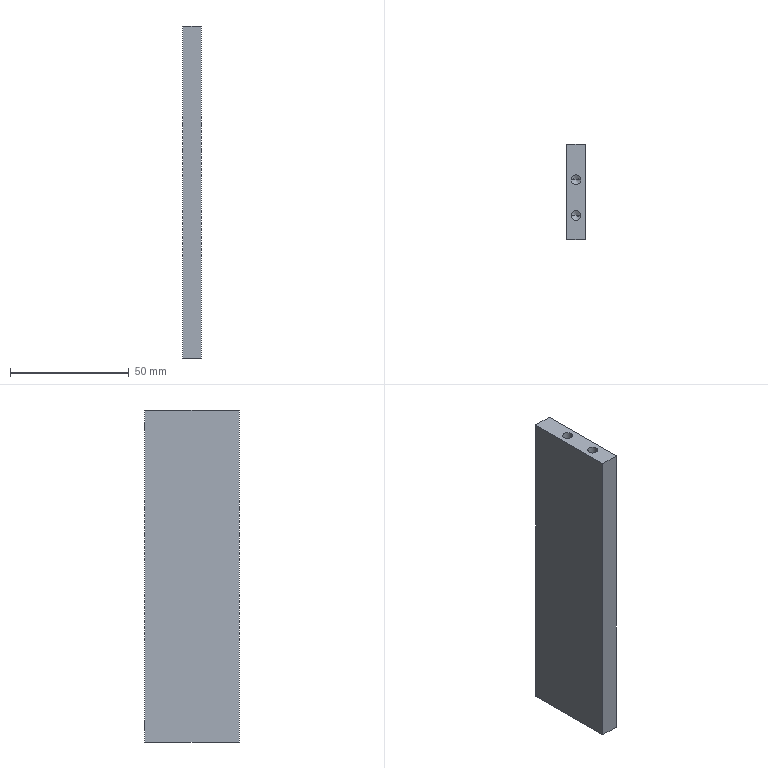Component | SolidWorks | FrameFrontMatchingPlate.1-1 | 1 solid | 30 faces | box 8 x 40 x 140 mm | volume 43911 mm3 | cylinder 12 | cone 12 | plane 6 | commonest cylinder face diameters 4.2 x8 3.3 x4
build123d program:
from build123d import *

# Parameters (mm, degrees)
SKETCH1_W             = 140
SKETCH1_H             = 40
BOSS_EXTRUDE1_DEPTH   = 8
M5_TAPPED_HOLE1_D     = 4.2
M5_TAPPED_HOLE1_DEPTH = 12.4
M5_TAPPED_HOLE1_TIP   = 1.262
M5_TAPPED_HOLE2_D     = 4.2
M5_TAPPED_HOLE2_DEPTH = 12.4
M5_TAPPED_HOLE2_TIP   = 1.262
M4_TAPPED_HOLE1_D     = 3.3
M4_TAPPED_HOLE1_DEPTH = 10.1
M4_TAPPED_HOLE1_TIP   = 0.9914


with BuildPart() as part:
    # Sketch1 → Boss-Extrude1 (new body)
    with BuildSketch(Plane.XY):
        Rectangle(SKETCH1_W, SKETCH1_H)
    extrude(amount=BOSS_EXTRUDE1_DEPTH)

    # M5 Tapped Hole1
    with Locations(Plane(origin=(70, 0, 0), x_dir=(0, 0, -1), z_dir=(1, 0, 0))):
        with Locations((-4, 5), (-4, -10)):
            Hole(M5_TAPPED_HOLE1_D / 2, depth=M5_TAPPED_HOLE1_DEPTH)
            with Locations((0, 0, -(M5_TAPPED_HOLE1_DEPTH + M5_TAPPED_HOLE1_TIP / 2))):  # 118° drill point
                Cone(0, M5_TAPPED_HOLE1_D / 2, M5_TAPPED_HOLE1_TIP, mode=Mode.SUBTRACT)

    # M5 Tapped Hole2
    with Locations(Plane.ZY.offset(70)):
        with Locations((4, 5), (4, -10)):
            Hole(M5_TAPPED_HOLE2_D / 2, depth=M5_TAPPED_HOLE2_DEPTH)
            with Locations((0, 0, -(M5_TAPPED_HOLE2_DEPTH + M5_TAPPED_HOLE2_TIP / 2))):  # 118° drill point
                Cone(0, M5_TAPPED_HOLE2_D / 2, M5_TAPPED_HOLE2_TIP, mode=Mode.SUBTRACT)

    # M4 Tapped Hole1
    with Locations(Plane(origin=(0, 20, 0), x_dir=(-1, 0, 0), z_dir=(0, 1, 0))):
        with Locations((63, 4), (-63, 4)):
            Hole(M4_TAPPED_HOLE1_D / 2, depth=M4_TAPPED_HOLE1_DEPTH)
            with Locations((0, 0, -(M4_TAPPED_HOLE1_DEPTH + M4_TAPPED_HOLE1_TIP / 2))):  # 118° drill point
                Cone(0, M4_TAPPED_HOLE1_D / 2, M4_TAPPED_HOLE1_TIP, mode=Mode.SUBTRACT)


solid = part.part

# Placed as in the assembly
solid = solid.moved(Location((13, 126.5, 0), (0, 90, 0)))
STEP:
#1=COLOUR_RGB('',0.7922,0.8196,0.9333);
#2=FILL_AREA_STYLE_COLOUR('',#1);
#3=FILL_AREA_STYLE('',(#2));
#4=SURFACE_STYLE_FILL_AREA(#3);
#5=SURFACE_SIDE_STYLE('',(#4));
#6=SURFACE_STYLE_USAGE(.BOTH.,#5);
#7=PRESENTATION_STYLE_ASSIGNMENT((#6));
#8=CARTESIAN_POINT('',(0.6043,5.37,2.48));
#9=VERTEX_POINT('',#8);
#10=CARTESIAN_POINT('',(0.7343,5.37,2.48));
#11=VERTEX_POINT('',#10);
#12=CARTESIAN_POINT('',(0.6693,5.37,2.48));
#13=DIRECTION('',(0.,1.,0.));
#14=DIRECTION('',(1.,0.,0.));
#15=AXIS2_PLACEMENT_3D('',#12,#13,#14);
#16=CIRCLE('',#15,0.06496);
#17=EDGE_CURVE('',#9,#11,#16,.T.);
#18=ORIENTED_EDGE('',*,*,#17,.F.);
#19=CARTESIAN_POINT('',(0.6043,5.768,2.48));
#20=VERTEX_POINT('',#19);
#21=CARTESIAN_POINT('',(0.6043,5.768,2.48));
#22=DIRECTION('',(0.,1.,0.));
#23=VECTOR('',#22,39.37);
#24=LINE('',#21,#23);
#25=EDGE_CURVE('',#9,#20,#24,.T.);
#26=ORIENTED_EDGE('',*,*,#25,.T.);
#27=CARTESIAN_POINT('',(0.7343,5.768,2.48));
#28=VERTEX_POINT('',#27);
#29=CARTESIAN_POINT('',(0.6693,5.768,2.48));
#30=DIRECTION('',(0.,1.,0.));
#31=DIRECTION('',(1.,0.,0.));
#32=AXIS2_PLACEMENT_3D('',#29,#30,#31);
#33=CIRCLE('',#32,0.06496);
#34=EDGE_CURVE('',#20,#28,#33,.T.);
#35=ORIENTED_EDGE('',*,*,#34,.T.);
#36=CARTESIAN_POINT('',(0.7343,5.768,2.48));
#37=DIRECTION('',(0.,1.,0.));
#38=VECTOR('',#37,39.37);
#39=LINE('',#36,#38);
#40=EDGE_CURVE('',#11,#28,#39,.T.);
#41=ORIENTED_EDGE('',*,*,#40,.F.);
#42=EDGE_LOOP('',(#18,#26,#35,#41));
#43=FACE_OUTER_BOUND('',#42,.T.);
#44=CARTESIAN_POINT('',(0.6693,5.768,2.48));
#45=DIRECTION('',(0.,1.,0.));
#46=DIRECTION('',(1.,0.,0.));
#47=AXIS2_PLACEMENT_3D('',#44,#45,#46);
#48=CYLINDRICAL_SURFACE('',#47,0.06496);
#49=ADVANCED_FACE('',(#43),#48,.F.);
#50=CARTESIAN_POINT('',(0.6693,5.331,2.48));
#51=VERTEX_POINT('',#50);
#52=CARTESIAN_POINT('',(0.7343,5.37,2.48));
#53=DIRECTION('',(0.8572,0.515,0.));
#54=VECTOR('',#53,39.37);
#55=LINE('',#52,#54);
#56=EDGE_CURVE('',#51,#11,#55,.T.);
#57=ORIENTED_EDGE('',*,*,#56,.F.);
#58=CARTESIAN_POINT('',(0.6043,5.37,2.48));
#59=DIRECTION('',(-0.8572,0.515,-0.));
#60=VECTOR('',#59,39.37);
#61=LINE('',#58,#60);
#62=EDGE_CURVE('',#51,#9,#61,.T.);
#63=ORIENTED_EDGE('',*,*,#62,.T.);
#64=ORIENTED_EDGE('',*,*,#17,.T.);
#65=EDGE_LOOP('',(#57,#63,#64));
#66=FACE_OUTER_BOUND('',#65,.T.);
#67=CARTESIAN_POINT('',(0.6693,5.37,2.48));
#68=DIRECTION('',(0.,1.,0.));
#69=DIRECTION('',(1.,0.,0.));
#70=AXIS2_PLACEMENT_3D('',#67,#68,#69);
#71=CONICAL_SURFACE('',#70,0.06496,1.03);
#72=ADVANCED_FACE('',(#66),#71,.F.);
#73=CARTESIAN_POINT('',(0.6043,5.37,-2.48));
#74=VERTEX_POINT('',#73);
#75=CARTESIAN_POINT('',(0.7343,5.37,-2.48));
#76=VERTEX_POINT('',#75);
#77=CARTESIAN_POINT('',(0.6693,5.37,-2.48));
#78=DIRECTION('',(0.,1.,0.));
#79=DIRECTION('',(1.,0.,0.));
#80=AXIS2_PLACEMENT_3D('',#77,#78,#79);
#81=CIRCLE('',#80,0.06496);
#82=EDGE_CURVE('',#74,#76,#81,.T.);
#83=ORIENTED_EDGE('',*,*,#82,.F.);
#84=CARTESIAN_POINT('',(0.6043,5.768,-2.48));
#85=VERTEX_POINT('',#84);
#86=CARTESIAN_POINT('',(0.6043,5.768,-2.48));
#87=DIRECTION('',(0.,1.,0.));
#88=VECTOR('',#87,39.37);
#89=LINE('',#86,#88);
#90=EDGE_CURVE('',#74,#85,#89,.T.);
#91=ORIENTED_EDGE('',*,*,#90,.T.);
#92=CARTESIAN_POINT('',(0.7343,5.768,-2.48));
#93=VERTEX_POINT('',#92);
#94=CARTESIAN_POINT('',(0.6693,5.768,-2.48));
#95=DIRECTION('',(0.,1.,0.));
#96=DIRECTION('',(1.,0.,0.));
#97=AXIS2_PLACEMENT_3D('',#94,#95,#96);
#98=CIRCLE('',#97,0.06496);
#99=EDGE_CURVE('',#85,#93,#98,.T.);
#100=ORIENTED_EDGE('',*,*,#99,.T.);
#101=CARTESIAN_POINT('',(0.7343,5.768,-2.48));
#102=DIRECTION('',(0.,1.,0.));
#103=VECTOR('',#102,39.37);
#104=LINE('',#101,#103);
#105=EDGE_CURVE('',#76,#93,#104,.T.);
#106=ORIENTED_EDGE('',*,*,#105,.F.);
#107=EDGE_LOOP('',(#83,#91,#100,#106));
#108=FACE_OUTER_BOUND('',#107,.T.);
#109=CARTESIAN_POINT('',(0.6693,5.768,-2.48));
#110=DIRECTION('',(0.,1.,0.));
#111=DIRECTION('',(1.,0.,0.));
#112=AXIS2_PLACEMENT_3D('',#109,#110,#111);
#113=CYLINDRICAL_SURFACE('',#112,0.06496);
#114=ADVANCED_FACE('',(#108),#113,.F.);
#115=CARTESIAN_POINT('',(0.6693,5.331,-2.48));
#116=VERTEX_POINT('',#115);
#117=CARTESIAN_POINT('',(0.7343,5.37,-2.48));
#118=DIRECTION('',(0.8572,0.515,0.));
#119=VECTOR('',#118,39.37);
#120=LINE('',#117,#119);
#121=EDGE_CURVE('',#116,#76,#120,.T.);
#122=ORIENTED_EDGE('',*,*,#121,.F.);
#123=CARTESIAN_POINT('',(0.6043,5.37,-2.48));
#124=DIRECTION('',(-0.8572,0.515,-0.));
#125=VECTOR('',#124,39.37);
#126=LINE('',#123,#125);
#127=EDGE_CURVE('',#116,#74,#126,.T.);
#128=ORIENTED_EDGE('',*,*,#127,.T.);
#129=ORIENTED_EDGE('',*,*,#82,.T.);
#130=EDGE_LOOP('',(#122,#128,#129));
#131=FACE_OUTER_BOUND('',#130,.T.);
#132=CARTESIAN_POINT('',(0.6693,5.37,-2.48));
#133=DIRECTION('',(0.,1.,0.));
#134=DIRECTION('',(1.,0.,0.));
#135=AXIS2_PLACEMENT_3D('',#132,#133,#134);
#136=CONICAL_SURFACE('',#135,0.06496,1.03);
#137=ADVANCED_FACE('',(#131),#136,.F.);
#138=CARTESIAN_POINT('',(0.5866,5.177,2.268));
#139=VERTEX_POINT('',#138);
#140=CARTESIAN_POINT('',(0.752,5.177,2.268));
#141=VERTEX_POINT('',#140);
#142=CARTESIAN_POINT('',(0.6693,5.177,2.268));
#143=DIRECTION('',(0.,0.,1.));
#144=DIRECTION('',(1.,0.,0.));
#145=AXIS2_PLACEMENT_3D('',#142,#143,#144);
#146=CIRCLE('',#145,0.08268);
#147=EDGE_CURVE('',#139,#141,#146,.T.);
#148=ORIENTED_EDGE('',*,*,#147,.F.);
#149=CARTESIAN_POINT('',(0.5866,5.177,2.756));
#150=VERTEX_POINT('',#149);
#151=CARTESIAN_POINT('',(0.5866,5.177,2.756));
#152=DIRECTION('',(0.,0.,1.));
#153=VECTOR('',#152,39.37);
#154=LINE('',#151,#153);
#155=EDGE_CURVE('',#139,#150,#154,.T.);
#156=ORIENTED_EDGE('',*,*,#155,.T.);
#157=CARTESIAN_POINT('',(0.752,5.177,2.756));
#158=VERTEX_POINT('',#157);
#159=CARTESIAN_POINT('',(0.6693,5.177,2.756));
#160=DIRECTION('',(0.,0.,1.));
#161=DIRECTION('',(1.,0.,0.));
#162=AXIS2_PLACEMENT_3D('',#159,#160,#161);
#163=CIRCLE('',#162,0.08268);
#164=EDGE_CURVE('',#150,#158,#163,.T.);
#165=ORIENTED_EDGE('',*,*,#164,.T.);
#166=CARTESIAN_POINT('',(0.752,5.177,2.756));
#167=DIRECTION('',(0.,0.,1.));
#168=VECTOR('',#167,39.37);
#169=LINE('',#166,#168);
#170=EDGE_CURVE('',#141,#158,#169,.T.);
#171=ORIENTED_EDGE('',*,*,#170,.F.);
#172=EDGE_LOOP('',(#148,#156,#165,#171));
#173=FACE_OUTER_BOUND('',#172,.T.);
#174=CARTESIAN_POINT('',(0.6693,5.177,2.756));
#175=DIRECTION('',(0.,0.,1.));
#176=DIRECTION('',(1.,0.,0.));
#177=AXIS2_PLACEMENT_3D('',#174,#175,#176);
#178=CYLINDRICAL_SURFACE('',#177,0.08268);
#179=ADVANCED_FACE('',(#173),#178,.F.);
#180=CARTESIAN_POINT('',(0.6693,5.177,2.218));
#181=VERTEX_POINT('',#180);
#182=CARTESIAN_POINT('',(0.752,5.177,2.268));
#183=DIRECTION('',(0.8572,0.,0.515));
#184=VECTOR('',#183,39.37);
#185=LINE('',#182,#184);
#186=EDGE_CURVE('',#181,#141,#185,.T.);
#187=ORIENTED_EDGE('',*,*,#186,.F.);
#188=CARTESIAN_POINT('',(0.5866,5.177,2.268));
#189=DIRECTION('',(-0.8572,0.,0.515));
#190=VECTOR('',#189,39.37);
#191=LINE('',#188,#190);
#192=EDGE_CURVE('',#181,#139,#191,.T.);
#193=ORIENTED_EDGE('',*,*,#192,.T.);
#194=ORIENTED_EDGE('',*,*,#147,.T.);
#195=EDGE_LOOP('',(#187,#193,#194));
#196=FACE_OUTER_BOUND('',#195,.T.);
#197=CARTESIAN_POINT('',(0.6693,5.177,2.268));
#198=DIRECTION('',(0.,0.,1.));
#199=DIRECTION('',(1.,0.,0.));
#200=AXIS2_PLACEMENT_3D('',#197,#198,#199);
#201=CONICAL_SURFACE('',#200,0.08268,1.03);
#202=ADVANCED_FACE('',(#196),#201,.F.);
#203=CARTESIAN_POINT('',(0.5866,4.587,2.268));
#204=VERTEX_POINT('',#203);
#205=CARTESIAN_POINT('',(0.752,4.587,2.268));
#206=VERTEX_POINT('',#205);
#207=CARTESIAN_POINT('',(0.6693,4.587,2.268));
#208=DIRECTION('',(0.,0.,1.));
#209=DIRECTION('',(1.,0.,0.));
#210=AXIS2_PLACEMENT_3D('',#207,#208,#209);
#211=CIRCLE('',#210,0.08268);
#212=EDGE_CURVE('',#204,#206,#211,.T.);
#213=ORIENTED_EDGE('',*,*,#212,.F.);
#214=CARTESIAN_POINT('',(0.5866,4.587,2.756));
#215=VERTEX_POINT('',#214);
#216=CARTESIAN_POINT('',(0.5866,4.587,2.756));
#217=DIRECTION('',(0.,0.,1.));
#218=VECTOR('',#217,39.37);
#219=LINE('',#216,#218);
#220=EDGE_CURVE('',#204,#215,#219,.T.);
#221=ORIENTED_EDGE('',*,*,#220,.T.);
#222=CARTESIAN_POINT('',(0.752,4.587,2.756));
#223=VERTEX_POINT('',#222);
#224=CARTESIAN_POINT('',(0.6693,4.587,2.756));
#225=DIRECTION('',(0.,0.,1.));
#226=DIRECTION('',(1.,0.,0.));
#227=AXIS2_PLACEMENT_3D('',#224,#225,#226);
#228=CIRCLE('',#227,0.08268);
#229=EDGE_CURVE('',#215,#223,#228,.T.);
#230=ORIENTED_EDGE('',*,*,#229,.T.);
#231=CARTESIAN_POINT('',(0.752,4.587,2.756));
#232=DIRECTION('',(0.,0.,1.));
#233=VECTOR('',#232,39.37);
#234=LINE('',#231,#233);
#235=EDGE_CURVE('',#206,#223,#234,.T.);
#236=ORIENTED_EDGE('',*,*,#235,.F.);
#237=EDGE_LOOP('',(#213,#221,#230,#236));
#238=FACE_OUTER_BOUND('',#237,.T.);
#239=CARTESIAN_POINT('',(0.6693,4.587,2.756));
#240=DIRECTION('',(0.,0.,1.));
#241=DIRECTION('',(1.,0.,0.));
#242=AXIS2_PLACEMENT_3D('',#239,#240,#241);
#243=CYLINDRICAL_SURFACE('',#242,0.08268);
#244=ADVANCED_FACE('',(#238),#243,.F.);
#245=CARTESIAN_POINT('',(0.6693,4.587,2.218));
#246=VERTEX_POINT('',#245);
#247=CARTESIAN_POINT('',(0.752,4.587,2.268));
#248=DIRECTION('',(0.8572,0.,0.515));
#249=VECTOR('',#248,39.37);
#250=LINE('',#247,#249);
#251=EDGE_CURVE('',#246,#206,#250,.T.);
#252=ORIENTED_EDGE('',*,*,#251,.F.);
#253=CARTESIAN_POINT('',(0.5866,4.587,2.268));
#254=DIRECTION('',(-0.8572,0.,0.515));
#255=VECTOR('',#254,39.37);
#256=LINE('',#253,#255);
#257=EDGE_CURVE('',#246,#204,#256,.T.);
#258=ORIENTED_EDGE('',*,*,#257,.T.);
#259=ORIENTED_EDGE('',*,*,#212,.T.);
#260=EDGE_LOOP('',(#252,#258,#259));
#261=FACE_OUTER_BOUND('',#260,.T.);
#262=CARTESIAN_POINT('',(0.6693,4.587,2.268));
#263=DIRECTION('',(0.,0.,1.));
#264=DIRECTION('',(1.,0.,0.));
#265=AXIS2_PLACEMENT_3D('',#262,#263,#264);
#266=CONICAL_SURFACE('',#265,0.08268,1.03);
#267=ADVANCED_FACE('',(#261),#266,.F.);
#268=CARTESIAN_POINT('',(0.752,5.177,-2.268));
#269=VERTEX_POINT('',#268);
#270=CARTESIAN_POINT('',(0.5866,5.177,-2.268));
#271=VERTEX_POINT('',#270);
#272=CARTESIAN_POINT('',(0.6693,5.177,-2.268));
#273=DIRECTION('',(0.,0.,-1.));
#274=DIRECTION('',(-1.,0.,0.));
#275=AXIS2_PLACEMENT_3D('',#272,#273,#274);
#276=CIRCLE('',#275,0.08268);
#277=EDGE_CURVE('',#269,#271,#276,.T.);
#278=ORIENTED_EDGE('',*,*,#277,.F.);
#279=CARTESIAN_POINT('',(0.752,5.177,-2.756));
#280=VERTEX_POINT('',#279);
#281=CARTESIAN_POINT('',(0.752,5.177,-2.756));
#282=DIRECTION('',(0.,0.,-1.));
#283=VECTOR('',#282,39.37);
#284=LINE('',#281,#283);
#285=EDGE_CURVE('',#269,#280,#284,.T.);
#286=ORIENTED_EDGE('',*,*,#285,.T.);
#287=CARTESIAN_POINT('',(0.5866,5.177,-2.756));
#288=VERTEX_POINT('',#287);
#289=CARTESIAN_POINT('',(0.6693,5.177,-2.756));
#290=DIRECTION('',(0.,0.,-1.));
#291=DIRECTION('',(-1.,0.,0.));
#292=AXIS2_PLACEMENT_3D('',#289,#290,#291);
#293=CIRCLE('',#292,0.08268);
#294=EDGE_CURVE('',#280,#288,#293,.T.);
#295=ORIENTED_EDGE('',*,*,#294,.T.);
#296=CARTESIAN_POINT('',(0.5866,5.177,-2.756));
#297=DIRECTION('',(0.,0.,-1.));
#298=VECTOR('',#297,39.37);
#299=LINE('',#296,#298);
#300=EDGE_CURVE('',#271,#288,#299,.T.);
#301=ORIENTED_EDGE('',*,*,#300,.F.);
#302=EDGE_LOOP('',(#278,#286,#295,#301));
#303=FACE_OUTER_BOUND('',#302,.T.);
#304=CARTESIAN_POINT('',(0.6693,5.177,-2.756));
#305=DIRECTION('',(0.,0.,-1.));
#306=DIRECTION('',(-1.,0.,0.));
#307=AXIS2_PLACEMENT_3D('',#304,#305,#306);
#308=CYLINDRICAL_SURFACE('',#307,0.08268);
#309=ADVANCED_FACE('',(#303),#308,.F.);
#310=CARTESIAN_POINT('',(0.6693,5.177,-2.218));
#311=VERTEX_POINT('',#310);
#312=CARTESIAN_POINT('',(0.5866,5.177,-2.268));
#313=DIRECTION('',(-0.8572,0.,-0.515));
#314=VECTOR('',#313,39.37);
#315=LINE('',#312,#314);
#316=EDGE_CURVE('',#311,#271,#315,.T.);
#317=ORIENTED_EDGE('',*,*,#316,.F.);
#318=CARTESIAN_POINT('',(0.752,5.177,-2.268));
#319=DIRECTION('',(0.8572,0.,-0.515));
#320=VECTOR('',#319,39.37);
#321=LINE('',#318,#320);
#322=EDGE_CURVE('',#311,#269,#321,.T.);
#323=ORIENTED_EDGE('',*,*,#322,.T.);
#324=ORIENTED_EDGE('',*,*,#277,.T.);
#325=EDGE_LOOP('',(#317,#323,#324));
#326=FACE_OUTER_BOUND('',#325,.T.);
#327=CARTESIAN_POINT('',(0.6693,5.177,-2.268));
#328=DIRECTION('',(0.,0.,-1.));
#329=DIRECTION('',(-1.,0.,0.));
#330=AXIS2_PLACEMENT_3D('',#327,#328,#329);
#331=CONICAL_SURFACE('',#330,0.08268,1.03);
#332=ADVANCED_FACE('',(#326),#331,.F.);
#333=CARTESIAN_POINT('',(0.752,4.587,-2.268));
#334=VERTEX_POINT('',#333);
#335=CARTESIAN_POINT('',(0.5866,4.587,-2.268));
#336=VERTEX_POINT('',#335);
#337=CARTESIAN_POINT('',(0.6693,4.587,-2.268));
#338=DIRECTION('',(0.,0.,-1.));
#339=DIRECTION('',(-1.,0.,0.));
#340=AXIS2_PLACEMENT_3D('',#337,#338,#339);
#341=CIRCLE('',#340,0.08268);
#342=EDGE_CURVE('',#334,#336,#341,.T.);
#343=ORIENTED_EDGE('',*,*,#342,.F.);
#344=CARTESIAN_POINT('',(0.752,4.587,-2.756));
#345=VERTEX_POINT('',#344);
#346=CARTESIAN_POINT('',(0.752,4.587,-2.756));
#347=DIRECTION('',(0.,0.,-1.));
#348=VECTOR('',#347,39.37);
#349=LINE('',#346,#348);
#350=EDGE_CURVE('',#334,#345,#349,.T.);
#351=ORIENTED_EDGE('',*,*,#350,.T.);
#352=CARTESIAN_POINT('',(0.5866,4.587,-2.756));
#353=VERTEX_POINT('',#352);
#354=CARTESIAN_POINT('',(0.6693,4.587,-2.756));
#355=DIRECTION('',(0.,0.,-1.));
#356=DIRECTION('',(-1.,0.,0.));
#357=AXIS2_PLACEMENT_3D('',#354,#355,#356);
#358=CIRCLE('',#357,0.08268);
#359=EDGE_CURVE('',#345,#353,#358,.T.);
#360=ORIENTED_EDGE('',*,*,#359,.T.);
#361=CARTESIAN_POINT('',(0.5866,4.587,-2.756));
#362=DIRECTION('',(0.,0.,-1.));
#363=VECTOR('',#362,39.37);
#364=LINE('',#361,#363);
#365=EDGE_CURVE('',#336,#353,#364,.T.);
#366=ORIENTED_EDGE('',*,*,#365,.F.);
#367=EDGE_LOOP('',(#343,#351,#360,#366));
#368=FACE_OUTER_BOUND('',#367,.T.);
#369=CARTESIAN_POINT('',(0.6693,4.587,-2.756));
#370=DIRECTION('',(0.,0.,-1.));
#371=DIRECTION('',(-1.,0.,0.));
#372=AXIS2_PLACEMENT_3D('',#369,#370,#371);
#373=CYLINDRICAL_SURFACE('',#372,0.08268);
#374=ADVANCED_FACE('',(#368),#373,.F.);
#375=CARTESIAN_POINT('',(0.6693,4.587,-2.218));
#376=VERTEX_POINT('',#375);
#377=CARTESIAN_POINT('',(0.5866,4.587,-2.268));
#378=DIRECTION('',(-0.8572,0.,-0.515));
#379=VECTOR('',#378,39.37);
#380=LINE('',#377,#379);
#381=EDGE_CURVE('',#376,#336,#380,.T.);
#382=ORIENTED_EDGE('',*,*,#381,.F.);
#383=CARTESIAN_POINT('',(0.752,4.587,-2.268));
#384=DIRECTION('',(0.8572,0.,-0.515));
#385=VECTOR('',#384,39.37);
#386=LINE('',#383,#385);
#387=EDGE_CURVE('',#376,#334,#386,.T.);
#388=ORIENTED_EDGE('',*,*,#387,.T.);
#389=ORIENTED_EDGE('',*,*,#342,.T.);
#390=EDGE_LOOP('',(#382,#388,#389));
#391=FACE_OUTER_BOUND('',#390,.T.);
#392=CARTESIAN_POINT('',(0.6693,4.587,-2.268));
#393=DIRECTION('',(0.,0.,-1.));
#394=DIRECTION('',(-1.,0.,0.));
#395=AXIS2_PLACEMENT_3D('',#392,#393,#394);
#396=CONICAL_SURFACE('',#395,0.08268,1.03);
#397=ADVANCED_FACE('',(#391),#396,.F.);
#398=CARTESIAN_POINT('',(0.6693,5.177,-2.756));
#399=DIRECTION('',(0.,0.,-1.));
#400=DIRECTION('',(-1.,0.,0.));
#401=AXIS2_PLACEMENT_3D('',#398,#399,#400);
#402=CIRCLE('',#401,0.08268);
#403=EDGE_CURVE('',#288,#280,#402,.T.);
#404=ORIENTED_EDGE('',*,*,#403,.F.);
#405=ORIENTED_EDGE('',*,*,#294,.F.);
#406=EDGE_LOOP('',(#404,#405));
#407=FACE_BOUND('',#406,.T.);
#408=CARTESIAN_POINT('',(0.6693,4.587,-2.756));
#409=DIRECTION('',(0.,0.,-1.));
#410=DIRECTION('',(-1.,0.,0.));
#411=AXIS2_PLACEMENT_3D('',#408,#409,#410);
#412=CIRCLE('',#411,0.08268);
#413=EDGE_CURVE('',#353,#345,#412,.T.);
#414=ORIENTED_EDGE('',*,*,#413,.F.);
#415=ORIENTED_EDGE('',*,*,#359,.F.);
#416=EDGE_LOOP('',(#414,#415));
#417=FACE_BOUND('',#416,.T.);
#418=CARTESIAN_POINT('',(0.5118,4.193,-2.756));
#419=VERTEX_POINT('',#418);
#420=CARTESIAN_POINT('',(0.5118,5.768,-2.756));
#421=VERTEX_POINT('',#420);
#422=CARTESIAN_POINT('',(0.5118,5.768,-2.756));
#423=DIRECTION('',(0.,1.,0.));
#424=VECTOR('',#423,39.37);
#425=LINE('',#422,#424);
#426=EDGE_CURVE('',#419,#421,#425,.T.);
#427=ORIENTED_EDGE('',*,*,#426,.T.);
#428=CARTESIAN_POINT('',(0.8268,5.768,-2.756));
#429=VERTEX_POINT('',#428);
#430=CARTESIAN_POINT('',(0.8268,5.768,-2.756));
#431=DIRECTION('',(-1.,0.,0.));
#432=VECTOR('',#431,39.37);
#433=LINE('',#430,#432);
#434=EDGE_CURVE('',#429,#421,#433,.T.);
#435=ORIENTED_EDGE('',*,*,#434,.F.);
#436=CARTESIAN_POINT('',(0.8268,4.193,-2.756));
#437=VERTEX_POINT('',#436);
#438=CARTESIAN_POINT('',(0.8268,5.768,-2.756));
#439=DIRECTION('',(0.,1.,0.));
#440=VECTOR('',#439,39.37);
#441=LINE('',#438,#440);
#442=EDGE_CURVE('',#437,#429,#441,.T.);
#443=ORIENTED_EDGE('',*,*,#442,.F.);
#444=CARTESIAN_POINT('',(0.8268,4.193,-2.756));
#445=DIRECTION('',(-1.,0.,0.));
#446=VECTOR('',#445,39.37);
#447=LINE('',#444,#446);
#448=EDGE_CURVE('',#437,#419,#447,.T.);
#449=ORIENTED_EDGE('',*,*,#448,.T.);
#450=EDGE_LOOP('',(#427,#435,#443,#449));
#451=FACE_OUTER_BOUND('',#450,.T.);
#452=CARTESIAN_POINT('',(0.8268,5.768,-2.756));
#453=DIRECTION('',(0.,0.,1.));
#454=DIRECTION('',(1.,0.,0.));
#455=AXIS2_PLACEMENT_3D('',#452,#453,#454);
#456=PLANE('',#455);
#457=ADVANCED_FACE('',(#407,#417,#451),#456,.F.);
#458=CARTESIAN_POINT('',(0.6693,5.768,2.48));
#459=DIRECTION('',(0.,1.,0.));
#460=DIRECTION('',(1.,0.,0.));
#461=AXIS2_PLACEMENT_3D('',#458,#459,#460);
#462=CIRCLE('',#461,0.06496);
#463=EDGE_CURVE('',#28,#20,#462,.T.);
#464=ORIENTED_EDGE('',*,*,#463,.F.);
#465=ORIENTED_EDGE('',*,*,#34,.F.);
#466=EDGE_LOOP('',(#464,#465));
#467=FACE_BOUND('',#466,.T.);
#468=CARTESIAN_POINT('',(0.6693,5.768,-2.48));
#469=DIRECTION('',(0.,1.,0.));
#470=DIRECTION('',(1.,0.,0.));
#471=AXIS2_PLACEMENT_3D('',#468,#469,#470);
#472=CIRCLE('',#471,0.06496);
#473=EDGE_CURVE('',#93,#85,#472,.T.);
#474=ORIENTED_EDGE('',*,*,#473,.F.);
#475=ORIENTED_EDGE('',*,*,#99,.F.);
#476=EDGE_LOOP('',(#474,#475));
#477=FACE_BOUND('',#476,.T.);
#478=CARTESIAN_POINT('',(0.5118,5.768,2.756));
#479=VERTEX_POINT('',#478);
#480=CARTESIAN_POINT('',(0.5118,5.768,2.756));
#481=DIRECTION('',(0.,0.,1.));
#482=VECTOR('',#481,39.37);
#483=LINE('',#480,#482);
#484=EDGE_CURVE('',#421,#479,#483,.T.);
#485=ORIENTED_EDGE('',*,*,#484,.T.);
#486=CARTESIAN_POINT('',(0.8268,5.768,2.756));
#487=VERTEX_POINT('',#486);
#488=CARTESIAN_POINT('',(0.8268,5.768,2.756));
#489=DIRECTION('',(-1.,0.,0.));
#490=VECTOR('',#489,39.37);
#491=LINE('',#488,#490);
#492=EDGE_CURVE('',#487,#479,#491,.T.);
#493=ORIENTED_EDGE('',*,*,#492,.F.);
#494=CARTESIAN_POINT('',(0.8268,5.768,2.756));
#495=DIRECTION('',(0.,0.,1.));
#496=VECTOR('',#495,39.37);
#497=LINE('',#494,#496);
#498=EDGE_CURVE('',#429,#487,#497,.T.);
#499=ORIENTED_EDGE('',*,*,#498,.F.);
#500=ORIENTED_EDGE('',*,*,#434,.T.);
#501=EDGE_LOOP('',(#485,#493,#499,#500));
#502=FACE_OUTER_BOUND('',#501,.T.);
#503=CARTESIAN_POINT('',(0.8268,5.768,2.756));
#504=DIRECTION('',(0.,-1.,0.));
#505=DIRECTION('',(-1.,0.,0.));
#506=AXIS2_PLACEMENT_3D('',#503,#504,#505);
#507=PLANE('',#506);
#508=ADVANCED_FACE('',(#467,#477,#502),#507,.F.);
#509=CARTESIAN_POINT('',(0.6693,5.177,2.756));
#510=DIRECTION('',(0.,0.,1.));
#511=DIRECTION('',(1.,0.,0.));
#512=AXIS2_PLACEMENT_3D('',#509,#510,#511);
#513=CIRCLE('',#512,0.08268);
#514=EDGE_CURVE('',#158,#150,#513,.T.);
#515=ORIENTED_EDGE('',*,*,#514,.F.);
#516=ORIENTED_EDGE('',*,*,#164,.F.);
#517=EDGE_LOOP('',(#515,#516));
#518=FACE_BOUND('',#517,.T.);
#519=CARTESIAN_POINT('',(0.6693,4.587,2.756));
#520=DIRECTION('',(0.,0.,1.));
#521=DIRECTION('',(1.,0.,0.));
#522=AXIS2_PLACEMENT_3D('',#519,#520,#521);
#523=CIRCLE('',#522,0.08268);
#524=EDGE_CURVE('',#223,#215,#523,.T.);
#525=ORIENTED_EDGE('',*,*,#524,.F.);
#526=ORIENTED_EDGE('',*,*,#229,.F.);
#527=EDGE_LOOP('',(#525,#526));
#528=FACE_BOUND('',#527,.T.);
#529=CARTESIAN_POINT('',(0.5118,4.193,2.756));
#530=VERTEX_POINT('',#529);
#531=CARTESIAN_POINT('',(0.5118,5.768,2.756));
#532=DIRECTION('',(0.,-1.,0.));
#533=VECTOR('',#532,39.37);
#534=LINE('',#531,#533);
#535=EDGE_CURVE('',#479,#530,#534,.T.);
#536=ORIENTED_EDGE('',*,*,#535,.T.);
#537=CARTESIAN_POINT('',(0.8268,4.193,2.756));
#538=VERTEX_POINT('',#537);
#539=CARTESIAN_POINT('',(0.8268,4.193,2.756));
#540=DIRECTION('',(-1.,0.,0.));
#541=VECTOR('',#540,39.37);
#542=LINE('',#539,#541);
#543=EDGE_CURVE('',#538,#530,#542,.T.);
#544=ORIENTED_EDGE('',*,*,#543,.F.);
#545=CARTESIAN_POINT('',(0.8268,5.768,2.756));
#546=DIRECTION('',(0.,-1.,0.));
#547=VECTOR('',#546,39.37);
#548=LINE('',#545,#547);
#549=EDGE_CURVE('',#487,#538,#548,.T.);
#550=ORIENTED_EDGE('',*,*,#549,.F.);
#551=ORIENTED_EDGE('',*,*,#492,.T.);
#552=EDGE_LOOP('',(#536,#544,#550,#551));
#553=FACE_OUTER_BOUND('',#552,.T.);
#554=CARTESIAN_POINT('',(0.8268,5.768,2.756));
#555=DIRECTION('',(0.,0.,-1.));
#556=DIRECTION('',(-1.,0.,0.));
#557=AXIS2_PLACEMENT_3D('',#554,#555,#556);
#558=PLANE('',#557);
#559=ADVANCED_FACE('',(#518,#528,#553),#558,.F.);
#560=CARTESIAN_POINT('',(0.5118,4.193,2.756));
#561=DIRECTION('',(0.,0.,-1.));
#562=VECTOR('',#561,39.37);
#563=LINE('',#560,#562);
#564=EDGE_CURVE('',#530,#419,#563,.T.);
#565=ORIENTED_EDGE('',*,*,#564,.T.);
#566=ORIENTED_EDGE('',*,*,#448,.F.);
#567=CARTESIAN_POINT('',(0.8268,4.193,2.756));
#568=DIRECTION('',(0.,0.,-1.));
#569=VECTOR('',#568,39.37);
#570=LINE('',#567,#569);
#571=EDGE_CURVE('',#538,#437,#570,.T.);
#572=ORIENTED_EDGE('',*,*,#571,.F.);
#573=ORIENTED_EDGE('',*,*,#543,.T.);
#574=EDGE_LOOP('',(#565,#566,#572,#573));
#575=FACE_OUTER_BOUND('',#574,.T.);
#576=CARTESIAN_POINT('',(0.8268,4.193,2.756));
#577=DIRECTION('',(0.,1.,0.));
#578=DIRECTION('',(1.,0.,0.));
#579=AXIS2_PLACEMENT_3D('',#576,#577,#578);
#580=PLANE('',#579);
#581=ADVANCED_FACE('',(#575),#580,.F.);
#582=ORIENTED_EDGE('',*,*,#442,.T.);
#583=ORIENTED_EDGE('',*,*,#498,.T.);
#584=ORIENTED_EDGE('',*,*,#549,.T.);
#585=ORIENTED_EDGE('',*,*,#571,.T.);
#586=EDGE_LOOP('',(#582,#583,#584,#585));
#587=FACE_OUTER_BOUND('',#586,.T.);
#588=CARTESIAN_POINT('',(0.8268,4.193,-2.756));
#589=DIRECTION('',(1.,0.,0.));
#590=DIRECTION('',(0.,0.,-1.));
#591=AXIS2_PLACEMENT_3D('',#588,#589,#590);
#592=PLANE('',#591);
#593=ADVANCED_FACE('',(#587),#592,.T.);
#594=ORIENTED_EDGE('',*,*,#426,.F.);
#595=ORIENTED_EDGE('',*,*,#564,.F.);
#596=ORIENTED_EDGE('',*,*,#535,.F.);
#597=ORIENTED_EDGE('',*,*,#484,.F.);
#598=EDGE_LOOP('',(#594,#595,#596,#597));
#599=FACE_OUTER_BOUND('',#598,.T.);
#600=CARTESIAN_POINT('',(0.5118,4.193,-2.756));
#601=DIRECTION('',(1.,0.,0.));
#602=DIRECTION('',(0.,0.,-1.));
#603=AXIS2_PLACEMENT_3D('',#600,#601,#602);
#604=PLANE('',#603);
#605=ADVANCED_FACE('',(#599),#604,.F.);
#606=ORIENTED_EDGE('',*,*,#387,.F.);
#607=ORIENTED_EDGE('',*,*,#381,.T.);
#608=CARTESIAN_POINT('',(0.6693,4.587,-2.268));
#609=DIRECTION('',(0.,0.,-1.));
#610=DIRECTION('',(-1.,0.,0.));
#611=AXIS2_PLACEMENT_3D('',#608,#609,#610);
#612=CIRCLE('',#611,0.08268);
#613=EDGE_CURVE('',#336,#334,#612,.T.);
#614=ORIENTED_EDGE('',*,*,#613,.T.);
#615=EDGE_LOOP('',(#606,#607,#614));
#616=FACE_OUTER_BOUND('',#615,.T.);
#617=CARTESIAN_POINT('',(0.6693,4.587,-2.268));
#618=DIRECTION('',(0.,0.,-1.));
#619=DIRECTION('',(-1.,0.,0.));
#620=AXIS2_PLACEMENT_3D('',#617,#618,#619);
#621=CONICAL_SURFACE('',#620,0.08268,1.03);
#622=ADVANCED_FACE('',(#616),#621,.F.);
#623=ORIENTED_EDGE('',*,*,#350,.F.);
#624=ORIENTED_EDGE('',*,*,#613,.F.);
#625=ORIENTED_EDGE('',*,*,#365,.T.);
#626=ORIENTED_EDGE('',*,*,#413,.T.);
#627=EDGE_LOOP('',(#623,#624,#625,#626));
#628=FACE_OUTER_BOUND('',#627,.T.);
#629=CARTESIAN_POINT('',(0.6693,4.587,-2.756));
#630=DIRECTION('',(0.,0.,-1.));
#631=DIRECTION('',(-1.,0.,0.));
#632=AXIS2_PLACEMENT_3D('',#629,#630,#631);
#633=CYLINDRICAL_SURFACE('',#632,0.08268);
#634=ADVANCED_FACE('',(#628),#633,.F.);
#635=ORIENTED_EDGE('',*,*,#322,.F.);
#636=ORIENTED_EDGE('',*,*,#316,.T.);
#637=CARTESIAN_POINT('',(0.6693,5.177,-2.268));
#638=DIRECTION('',(0.,0.,-1.));
#639=DIRECTION('',(-1.,0.,0.));
#640=AXIS2_PLACEMENT_3D('',#637,#638,#639);
#641=CIRCLE('',#640,0.08268);
#642=EDGE_CURVE('',#271,#269,#641,.T.);
#643=ORIENTED_EDGE('',*,*,#642,.T.);
#644=EDGE_LOOP('',(#635,#636,#643));
#645=FACE_OUTER_BOUND('',#644,.T.);
#646=CARTESIAN_POINT('',(0.6693,5.177,-2.268));
#647=DIRECTION('',(0.,0.,-1.));
#648=DIRECTION('',(-1.,0.,0.));
#649=AXIS2_PLACEMENT_3D('',#646,#647,#648);
#650=CONICAL_SURFACE('',#649,0.08268,1.03);
#651=ADVANCED_FACE('',(#645),#650,.F.);
#652=ORIENTED_EDGE('',*,*,#285,.F.);
#653=ORIENTED_EDGE('',*,*,#642,.F.);
#654=ORIENTED_EDGE('',*,*,#300,.T.);
#655=ORIENTED_EDGE('',*,*,#403,.T.);
#656=EDGE_LOOP('',(#652,#653,#654,#655));
#657=FACE_OUTER_BOUND('',#656,.T.);
#658=CARTESIAN_POINT('',(0.6693,5.177,-2.756));
#659=DIRECTION('',(0.,0.,-1.));
#660=DIRECTION('',(-1.,0.,0.));
#661=AXIS2_PLACEMENT_3D('',#658,#659,#660);
#662=CYLINDRICAL_SURFACE('',#661,0.08268);
#663=ADVANCED_FACE('',(#657),#662,.F.);
#664=ORIENTED_EDGE('',*,*,#257,.F.);
#665=ORIENTED_EDGE('',*,*,#251,.T.);
#666=CARTESIAN_POINT('',(0.6693,4.587,2.268));
#667=DIRECTION('',(0.,0.,1.));
#668=DIRECTION('',(1.,0.,0.));
#669=AXIS2_PLACEMENT_3D('',#666,#667,#668);
#670=CIRCLE('',#669,0.08268);
#671=EDGE_CURVE('',#206,#204,#670,.T.);
#672=ORIENTED_EDGE('',*,*,#671,.T.);
#673=EDGE_LOOP('',(#664,#665,#672));
#674=FACE_OUTER_BOUND('',#673,.T.);
#675=CARTESIAN_POINT('',(0.6693,4.587,2.268));
#676=DIRECTION('',(0.,0.,1.));
#677=DIRECTION('',(1.,0.,0.));
#678=AXIS2_PLACEMENT_3D('',#675,#676,#677);
#679=CONICAL_SURFACE('',#678,0.08268,1.03);
#680=ADVANCED_FACE('',(#674),#679,.F.);
#681=ORIENTED_EDGE('',*,*,#220,.F.);
#682=ORIENTED_EDGE('',*,*,#671,.F.);
#683=ORIENTED_EDGE('',*,*,#235,.T.);
#684=ORIENTED_EDGE('',*,*,#524,.T.);
#685=EDGE_LOOP('',(#681,#682,#683,#684));
#686=FACE_OUTER_BOUND('',#685,.T.);
#687=CARTESIAN_POINT('',(0.6693,4.587,2.756));
#688=DIRECTION('',(0.,0.,1.));
#689=DIRECTION('',(1.,0.,0.));
#690=AXIS2_PLACEMENT_3D('',#687,#688,#689);
#691=CYLINDRICAL_SURFACE('',#690,0.08268);
#692=ADVANCED_FACE('',(#686),#691,.F.);
#693=ORIENTED_EDGE('',*,*,#192,.F.);
#694=ORIENTED_EDGE('',*,*,#186,.T.);
#695=CARTESIAN_POINT('',(0.6693,5.177,2.268));
#696=DIRECTION('',(0.,0.,1.));
#697=DIRECTION('',(1.,0.,0.));
#698=AXIS2_PLACEMENT_3D('',#695,#696,#697);
#699=CIRCLE('',#698,0.08268);
#700=EDGE_CURVE('',#141,#139,#699,.T.);
#701=ORIENTED_EDGE('',*,*,#700,.T.);
#702=EDGE_LOOP('',(#693,#694,#701));
#703=FACE_OUTER_BOUND('',#702,.T.);
#704=CARTESIAN_POINT('',(0.6693,5.177,2.268));
#705=DIRECTION('',(0.,0.,1.));
#706=DIRECTION('',(1.,0.,0.));
#707=AXIS2_PLACEMENT_3D('',#704,#705,#706);
#708=CONICAL_SURFACE('',#707,0.08268,1.03);
#709=ADVANCED_FACE('',(#703),#708,.F.);
#710=ORIENTED_EDGE('',*,*,#155,.F.);
#711=ORIENTED_EDGE('',*,*,#700,.F.);
#712=ORIENTED_EDGE('',*,*,#170,.T.);
#713=ORIENTED_EDGE('',*,*,#514,.T.);
#714=EDGE_LOOP('',(#710,#711,#712,#713));
#715=FACE_OUTER_BOUND('',#714,.T.);
#716=CARTESIAN_POINT('',(0.6693,5.177,2.756));
#717=DIRECTION('',(0.,0.,1.));
#718=DIRECTION('',(1.,0.,0.));
#719=AXIS2_PLACEMENT_3D('',#716,#717,#718);
#720=CYLINDRICAL_SURFACE('',#719,0.08268);
#721=ADVANCED_FACE('',(#715),#720,.F.);
#722=ORIENTED_EDGE('',*,*,#127,.F.);
#723=ORIENTED_EDGE('',*,*,#121,.T.);
#724=CARTESIAN_POINT('',(0.6693,5.37,-2.48));
#725=DIRECTION('',(0.,1.,0.));
#726=DIRECTION('',(1.,0.,0.));
#727=AXIS2_PLACEMENT_3D('',#724,#725,#726);
#728=CIRCLE('',#727,0.06496);
#729=EDGE_CURVE('',#76,#74,#728,.T.);
#730=ORIENTED_EDGE('',*,*,#729,.T.);
#731=EDGE_LOOP('',(#722,#723,#730));
#732=FACE_OUTER_BOUND('',#731,.T.);
#733=CARTESIAN_POINT('',(0.6693,5.37,-2.48));
#734=DIRECTION('',(0.,1.,0.));
#735=DIRECTION('',(1.,0.,0.));
#736=AXIS2_PLACEMENT_3D('',#733,#734,#735);
#737=CONICAL_SURFACE('',#736,0.06496,1.03);
#738=ADVANCED_FACE('',(#732),#737,.F.);
#739=ORIENTED_EDGE('',*,*,#90,.F.);
#740=ORIENTED_EDGE('',*,*,#729,.F.);
#741=ORIENTED_EDGE('',*,*,#105,.T.);
#742=ORIENTED_EDGE('',*,*,#473,.T.);
#743=EDGE_LOOP('',(#739,#740,#741,#742));
#744=FACE_OUTER_BOUND('',#743,.T.);
#745=CARTESIAN_POINT('',(0.6693,5.768,-2.48));
#746=DIRECTION('',(0.,1.,0.));
#747=DIRECTION('',(1.,0.,0.));
#748=AXIS2_PLACEMENT_3D('',#745,#746,#747);
#749=CYLINDRICAL_SURFACE('',#748,0.06496);
#750=ADVANCED_FACE('',(#744),#749,.F.);
#751=ORIENTED_EDGE('',*,*,#62,.F.);
#752=ORIENTED_EDGE('',*,*,#56,.T.);
#753=CARTESIAN_POINT('',(0.6693,5.37,2.48));
#754=DIRECTION('',(0.,1.,0.));
#755=DIRECTION('',(1.,0.,0.));
#756=AXIS2_PLACEMENT_3D('',#753,#754,#755);
#757=CIRCLE('',#756,0.06496);
#758=EDGE_CURVE('',#11,#9,#757,.T.);
#759=ORIENTED_EDGE('',*,*,#758,.T.);
#760=EDGE_LOOP('',(#751,#752,#759));
#761=FACE_OUTER_BOUND('',#760,.T.);
#762=CARTESIAN_POINT('',(0.6693,5.37,2.48));
#763=DIRECTION('',(0.,1.,0.));
#764=DIRECTION('',(1.,0.,0.));
#765=AXIS2_PLACEMENT_3D('',#762,#763,#764);
#766=CONICAL_SURFACE('',#765,0.06496,1.03);
#767=ADVANCED_FACE('',(#761),#766,.F.);
#768=ORIENTED_EDGE('',*,*,#25,.F.);
#769=ORIENTED_EDGE('',*,*,#758,.F.);
#770=ORIENTED_EDGE('',*,*,#40,.T.);
#771=ORIENTED_EDGE('',*,*,#463,.T.);
#772=EDGE_LOOP('',(#768,#769,#770,#771));
#773=FACE_OUTER_BOUND('',#772,.T.);
#774=CARTESIAN_POINT('',(0.6693,5.768,2.48));
#775=DIRECTION('',(0.,1.,0.));
#776=DIRECTION('',(1.,0.,0.));
#777=AXIS2_PLACEMENT_3D('',#774,#775,#776);
#778=CYLINDRICAL_SURFACE('',#777,0.06496);
#779=ADVANCED_FACE('',(#773),#778,.F.);
#780=CLOSED_SHELL('',(#49,#72,#114,#137,#179,#202,#244,#267,#309,#332,#374,#397,#457,#508,#559,#581,#593,#605,#622,#634,#651,#663,#680,#692,#709,#721,#738,#750,#767,#779));
#781=MANIFOLD_SOLID_BREP('',#780);
#782=STYLED_ITEM('',(#7),#781);
#783=(LENGTH_UNIT()NAMED_UNIT(*)SI_UNIT($,.METRE.));
#784=LENGTH_MEASURE_WITH_UNIT(LENGTH_MEASURE(0.0254),#783);
#785=DIMENSIONAL_EXPONENTS(1.,0.,0.,0.,0.,0.,0.);
#786=(CONVERSION_BASED_UNIT('',#784)LENGTH_UNIT()NAMED_UNIT(#785));
#787=UNCERTAINTY_MEASURE_WITH_UNIT(LENGTH_MEASURE(0.00001),#786,'','');
#788=(NAMED_UNIT(*)PLANE_ANGLE_UNIT()SI_UNIT($,.RADIAN.));
#789=(NAMED_UNIT(*)SI_UNIT($,.STERADIAN.)SOLID_ANGLE_UNIT());
#790=(GEOMETRIC_REPRESENTATION_CONTEXT(3)GLOBAL_UNCERTAINTY_ASSIGNED_CONTEXT((#787))GLOBAL_UNIT_ASSIGNED_CONTEXT((#786,#788,#789))REPRESENTATION_CONTEXT('',''));
#791=MECHANICAL_DESIGN_GEOMETRIC_PRESENTATION_REPRESENTATION('',(#782),#790);
#792=CARTESIAN_POINT('',(0.,0.,0.));
#793=DIRECTION('',(0.,0.,1.));
#794=DIRECTION('',(1.,0.,0.));
#795=AXIS2_PLACEMENT_3D('',#792,#793,#794);
#796=(LENGTH_UNIT()NAMED_UNIT(*)SI_UNIT($,.METRE.));
#797=LENGTH_MEASURE_WITH_UNIT(LENGTH_MEASURE(0.0254),#796);
#798=DIMENSIONAL_EXPONENTS(1.,0.,0.,0.,0.,0.,0.);
#799=(CONVERSION_BASED_UNIT('',#797)LENGTH_UNIT()NAMED_UNIT(#798));
#800=UNCERTAINTY_MEASURE_WITH_UNIT(LENGTH_MEASURE(0.00001),#799,'','');
#801=(NAMED_UNIT(*)PLANE_ANGLE_UNIT()SI_UNIT($,.RADIAN.));
#802=(NAMED_UNIT(*)SI_UNIT($,.STERADIAN.)SOLID_ANGLE_UNIT());
#803=(GEOMETRIC_REPRESENTATION_CONTEXT(3)GLOBAL_UNCERTAINTY_ASSIGNED_CONTEXT((#800))GLOBAL_UNIT_ASSIGNED_CONTEXT((#799,#801,#802))REPRESENTATION_CONTEXT('',''));
#804=ADVANCED_BREP_SHAPE_REPRESENTATION('',(#781,#795),#803);
#805=PRESENTATION_LAYER_ASSIGNMENT('','',(#782));